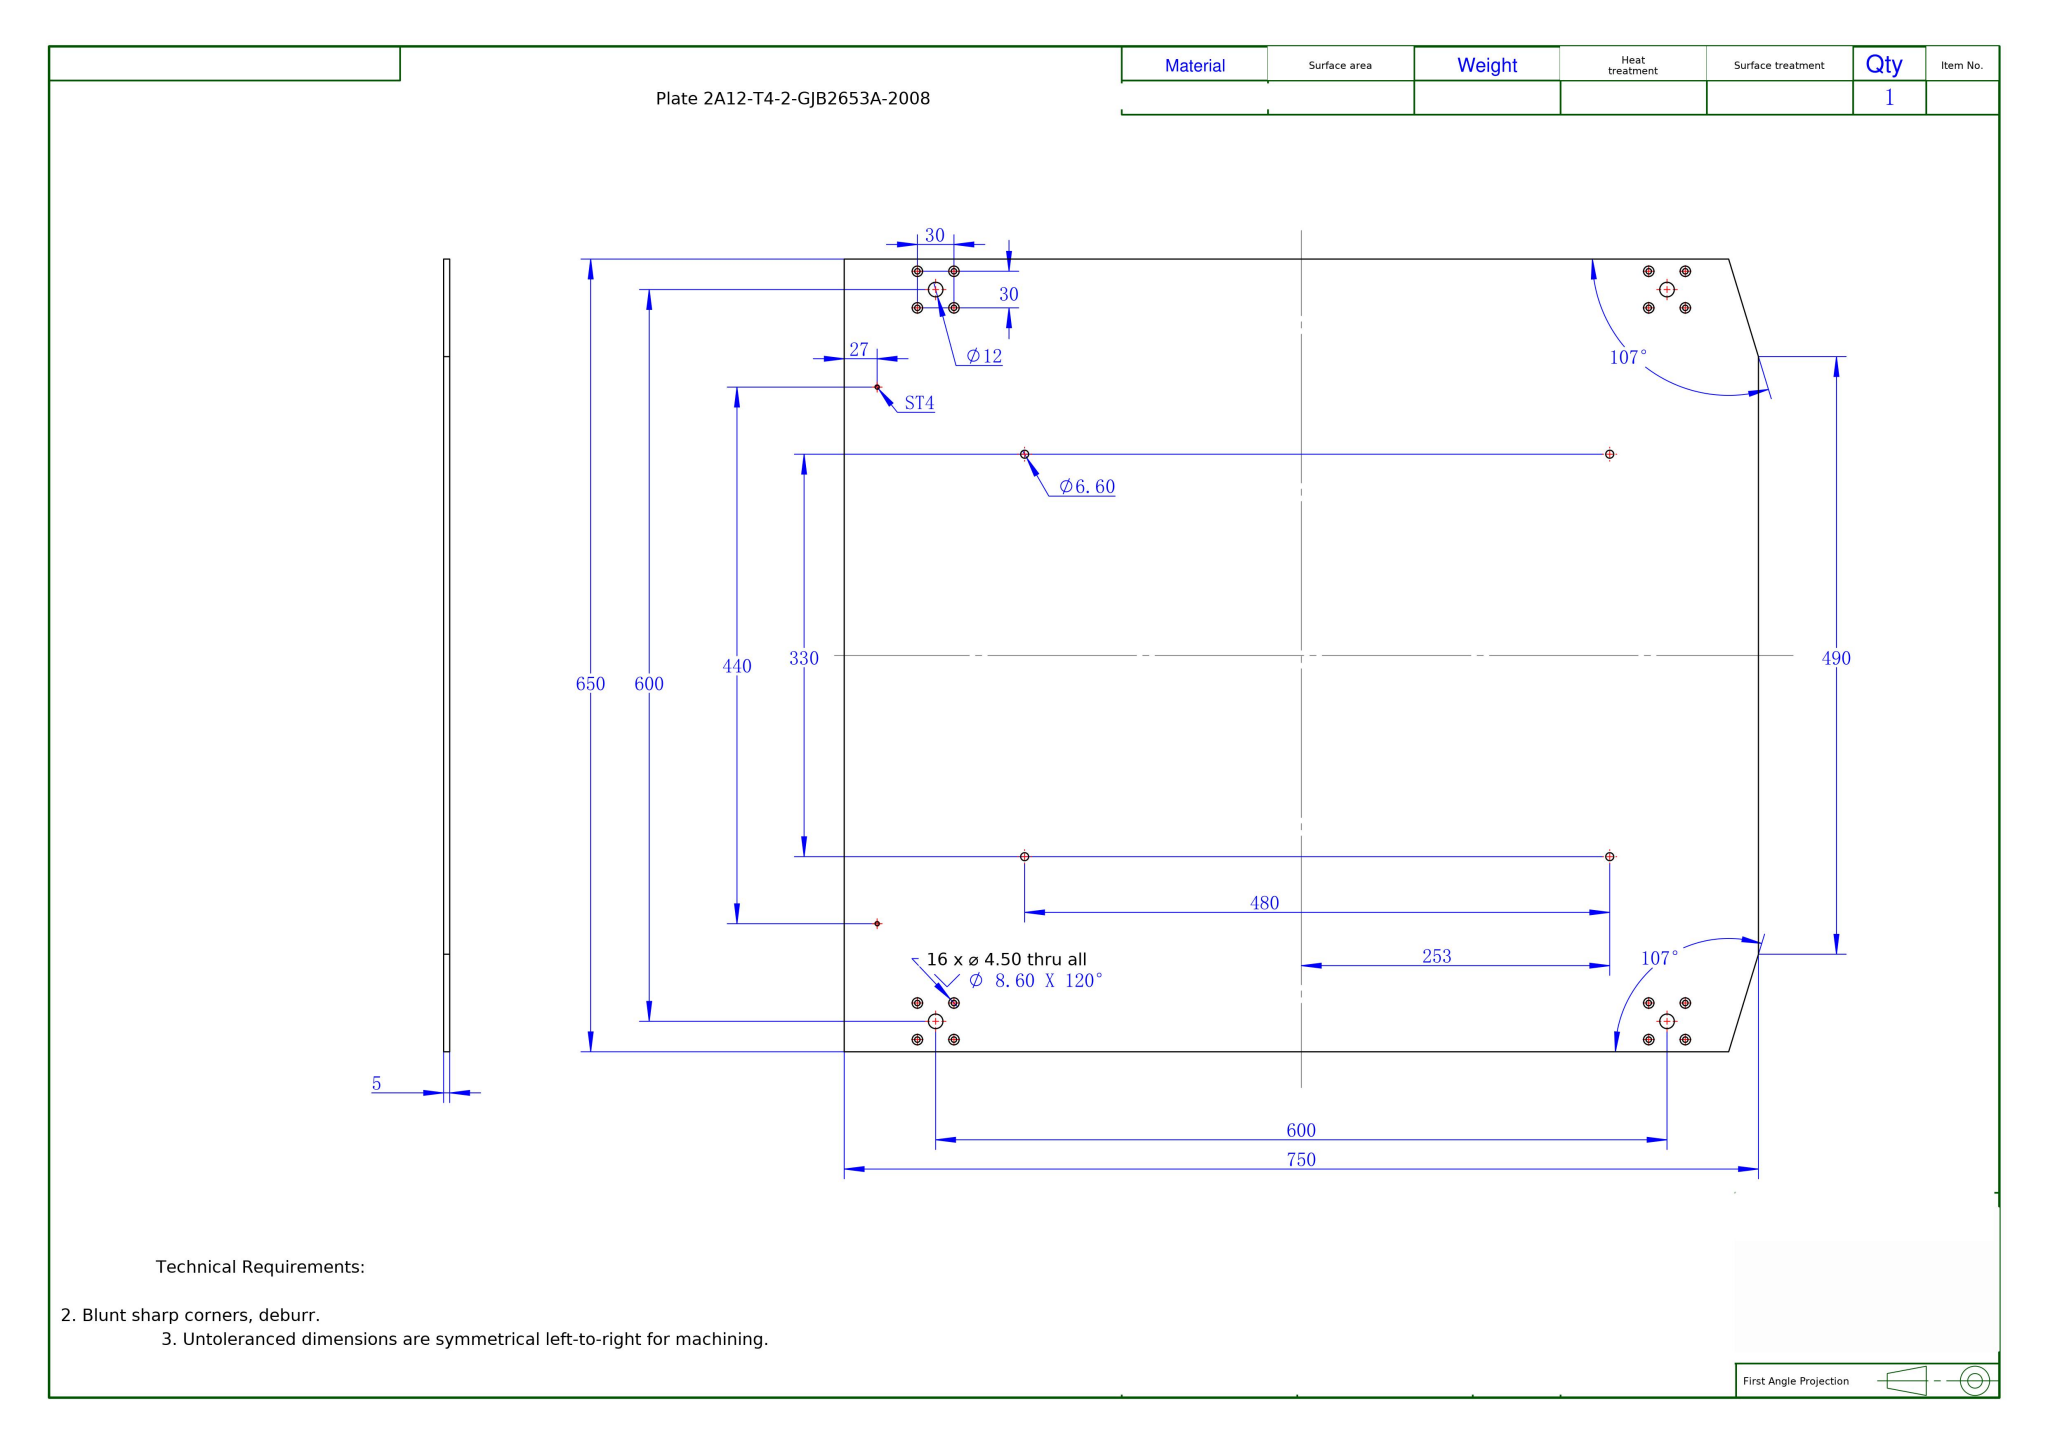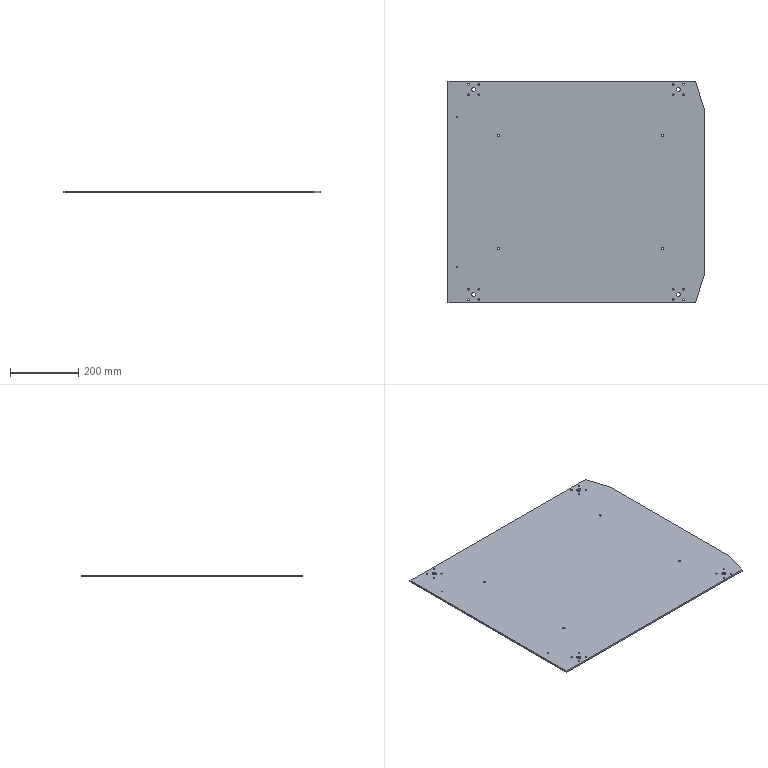Part | SolidWorks | mm | material Plate 2A12-T4-2-GJB2653A-2008 | 1 solid | 92 faces | box 750 x 650 x 5 mm | volume 2423055 mm3 | cylinder 52 | cone 32 | plane 8 | commonest cylinder face diameters 4.5 x32 6.6 x8 12 x8 3.3 x4